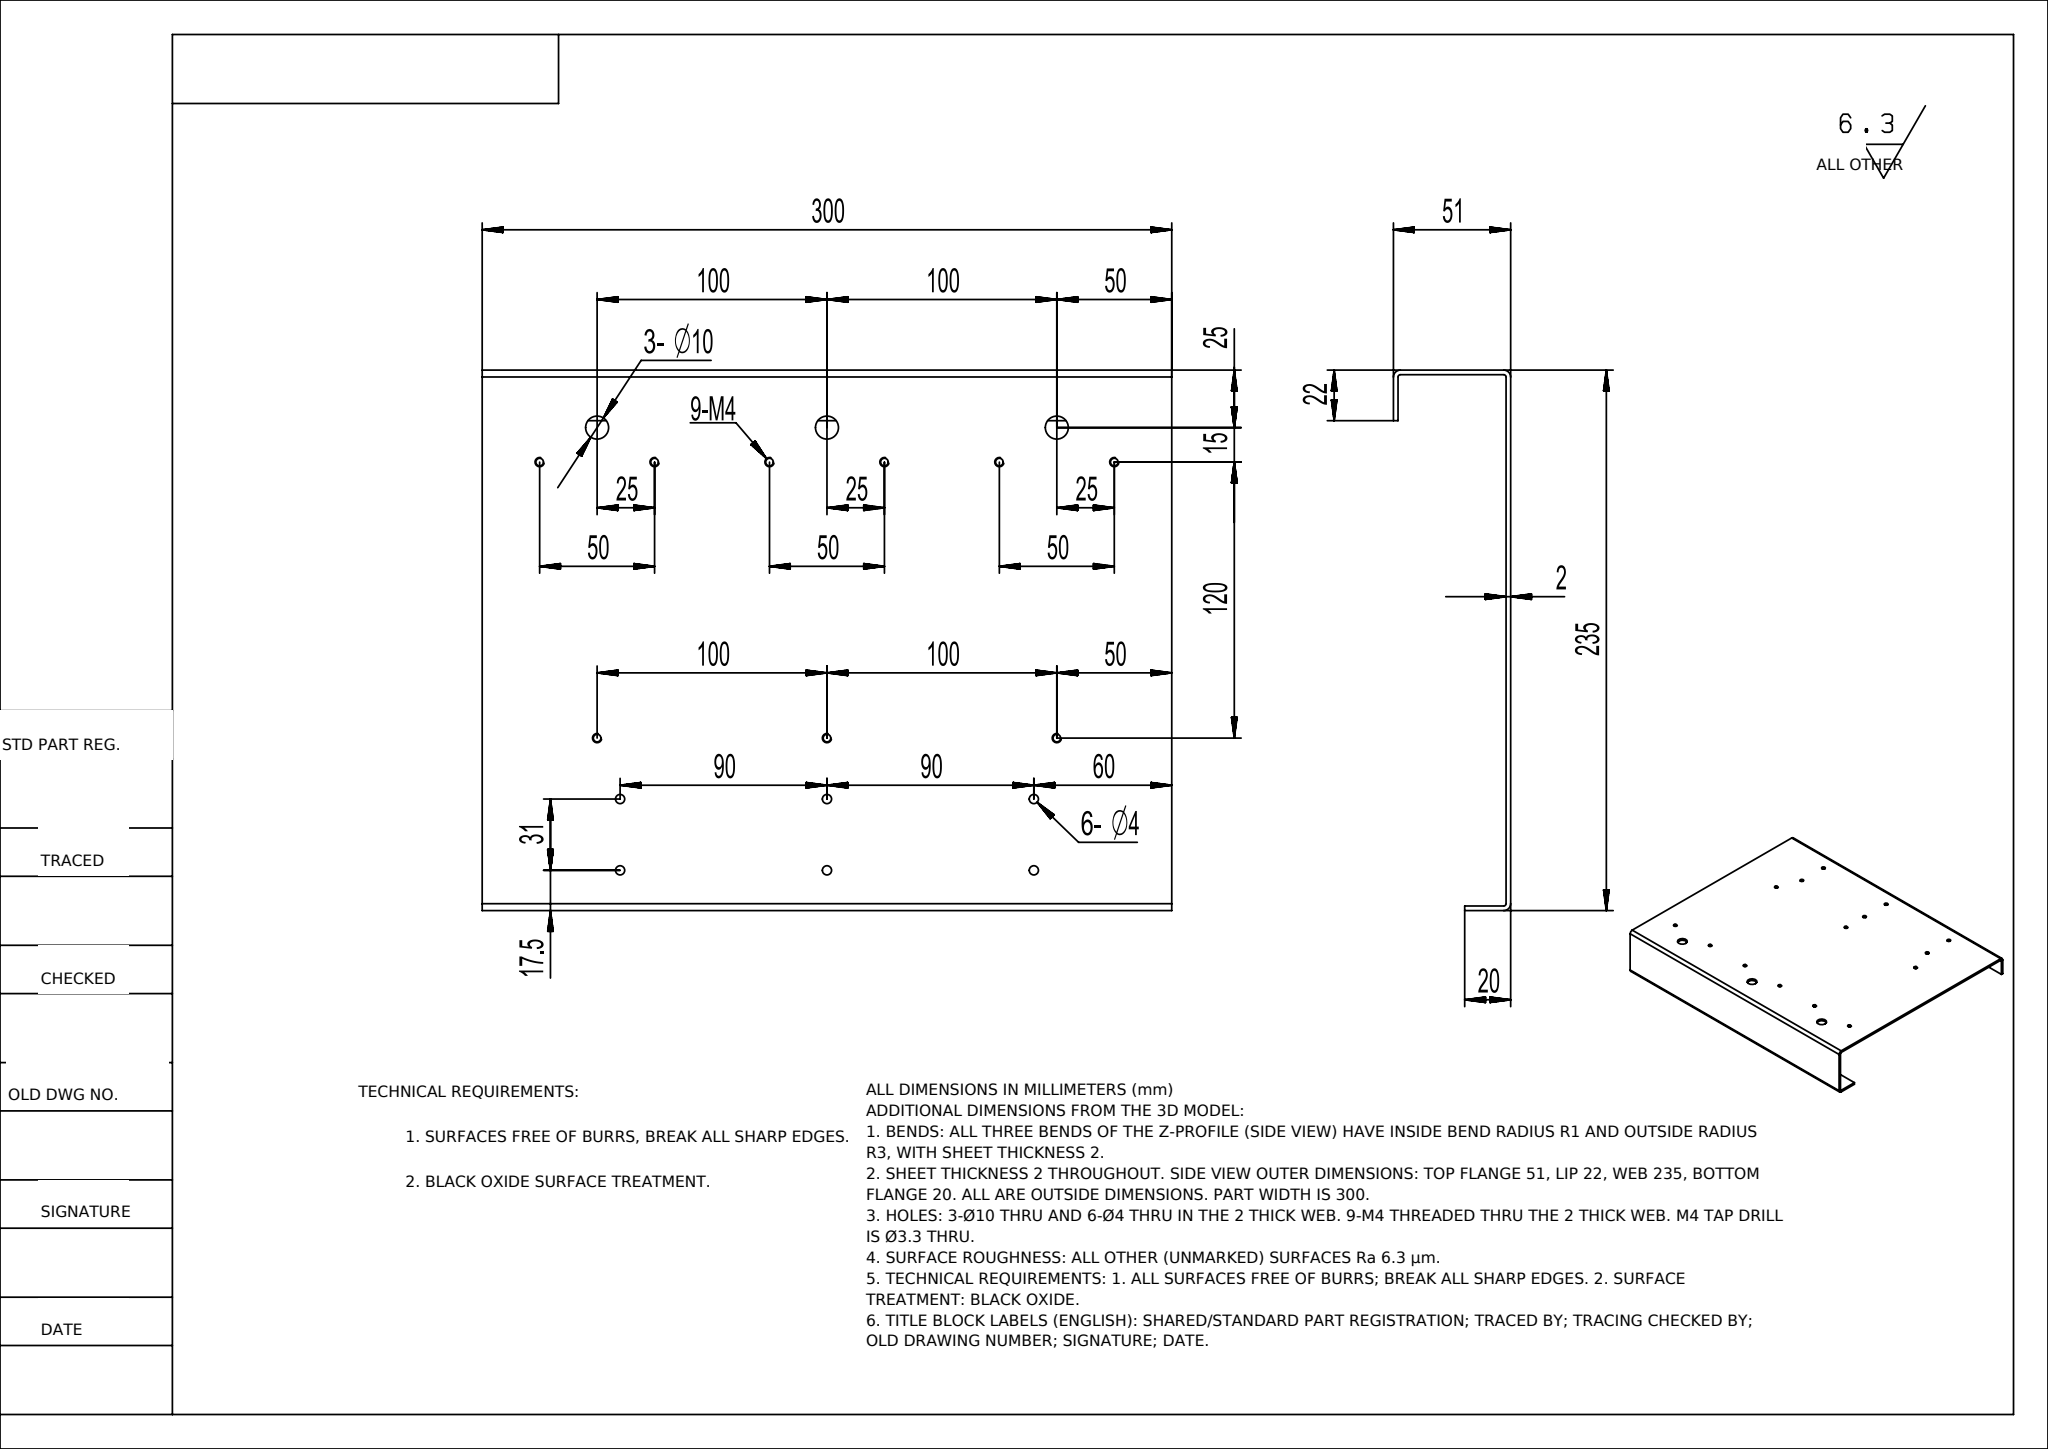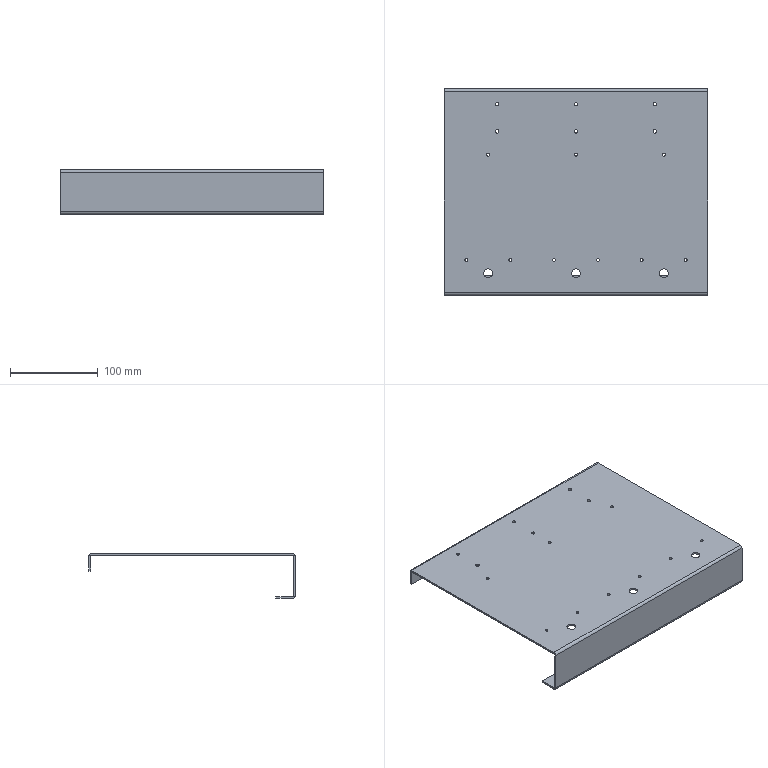Part | NX | mm | 1 solid | 36 faces | box 300 x 235 x 51 mm | volume 190879 mm3 | cylinder 24 | plane 12 | commonest cylinder face diameters 3.3 x9 4 x6 6 x3 2 x3 10 x3